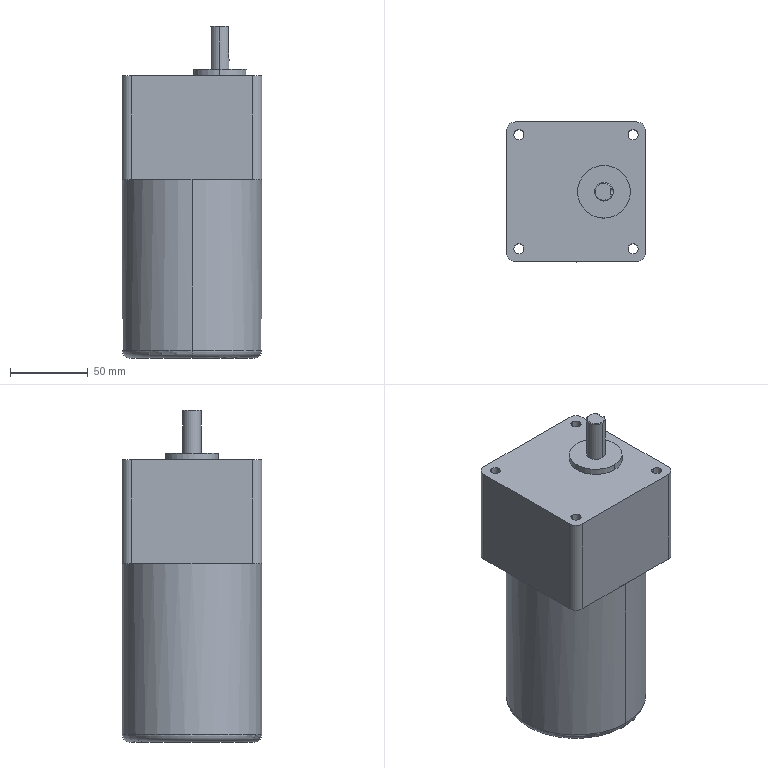Component | SolidWorks | LD101-02-5IK60Q1-C-5GN180K-1 | 1 solid | 39 faces | box 90 x 90 x 214 mm | volume 1268487 mm3 | cylinder 19 | plane 15 | cone 3 | torus 2 | commonest cylinder face diameters 6.5 x8 12 x6 34 x2 90 x2 4 x1 | material SUS304
build123d program:
from build123d import *

# Parameters (mm, degrees)
BOSS_EXTRUDE1_DEPTH        = 7
SKETCH2_R                  = 45
BOSS_EXTRUDE2_DEPTH        = 122
FILLET1_R                  = 5
BOSS_EXTRUDE3_START        = 60
BOSS_EXTRUDE3_DEPTH        = 60
SKETCH4_R                  = 17
BOSS_EXTRUDE4_DEPTH        = 4
SKETCH5_R                  = 6
BOSS_EXTRUDE5_DEPTH        = 32
CHAMFER1_SIZE              = 0.5
F_6_5_6_5_DIAMETER_HOLE1_D = 6.5
CUT_EXTRUDE2_START         = 24
CUT_EXTRUDE2_DEPTH         = 2


with BuildPart() as part:
    # Sketch1 → Boss-Extrude1 (new body)
    with BuildSketch(Plane(origin=(0, 0, 0), x_dir=(0, 0, -1), z_dir=(1, 0, 0))):
        with BuildLine():
            Line((-39, -45), (39, -45))
            ThreePointArc((39, -45), (43.243, -43.243), (45, -39))
            Line((45, -39), (45, 39))
            ThreePointArc((45, 39), (43.243, 43.243), (39, 45))
            Line((39, 45), (-39, 45))
            ThreePointArc((-39, 45), (-43.243, 43.243), (-45, 39))
            Line((-45, 39), (-45, -39))
            ThreePointArc((-45, -39), (-43.243, -43.243), (-39, -45))
        make_face()
    extrude(amount=-BOSS_EXTRUDE1_DEPTH)

    # Sketch2 → Boss-Extrude2 (add)
    with BuildSketch(Plane(origin=(0, 0, 0), x_dir=(0, 0, -1), z_dir=(1, 0, 0))):
        Circle(SKETCH2_R)
    extrude(amount=-BOSS_EXTRUDE2_DEPTH)

    # Fillet1
    fillet1_edges = [part.edges().sort_by_distance(p)[0] for p in [
        (-122, 0, 45),
    ]]
    fillet(fillet1_edges, radius=FILLET1_R)

    # Sketch3 → Boss-Extrude3 (add)
    with BuildSketch(Plane(origin=(0, 0, 0), x_dir=(0, 0, -1), z_dir=(1, 0, 0)).offset(BOSS_EXTRUDE3_START)):
        with BuildLine():
            Line((45, -39), (45, 39))
            ThreePointArc((45, 39), (43.243, 43.243), (39, 45))
            Line((39, 45), (-39, 45))
            ThreePointArc((-39, 45), (-43.243, 43.243), (-45, 39))
            Line((-45, 39), (-45, -39))
            ThreePointArc((-45, -39), (-43.243, -43.243), (-39, -45))
            Line((-39, -45), (39, -45))
            ThreePointArc((39, -45), (43.243, -43.243), (45, -39))
        make_face()
    extrude(amount=-BOSS_EXTRUDE3_DEPTH)

    # Sketch4 → Boss-Extrude4 (add)
    with BuildSketch(Plane(origin=(60, 0, 0), x_dir=(0, 0, -1), z_dir=(1, 0, 0))):
        with Locations((0, 18)):
            Circle(SKETCH4_R)
    extrude(amount=BOSS_EXTRUDE4_DEPTH)

    # Sketch5 → Boss-Extrude5 (add)
    with BuildSketch(Plane(origin=(60, 0, 0), x_dir=(0, 0, -1), z_dir=(1, 0, 0))):
        with Locations((0, 18)):
            Circle(SKETCH5_R)
    extrude(amount=BOSS_EXTRUDE5_DEPTH)

    # Chamfer1
    chamfer1_edges = [part.edges().sort_by_distance(p)[0] for p in [
        (92, 18, 6),
    ]]
    chamfer(chamfer1_edges, length=CHAMFER1_SIZE)

    # 6.5 _6.5_ Diameter Hole1 (through all)
    with Locations(Plane(origin=(60, 0, 0), x_dir=(0, 0, -1), z_dir=(1, 0, 0))):
        with Locations((36.77, 36.77), (36.77, -36.77), (-36.77, -36.77), (-36.77, 36.77)):
            Hole(F_6_5_6_5_DIAMETER_HOLE1_D / 2)

    # Sketch12 → Cut-Extrude2 (cut)
    with BuildSketch(Plane(origin=(0, 0, 0), x_dir=(1, 0, 0), z_dir=(0, 1, 0)).offset(CUT_EXTRUDE2_START)):
        with BuildLine():
            Line((92, -2), (72, -2))
            ThreePointArc((72, -2), (70, 0), (72, 2))
            Line((72, 2), (92, 2))
            ThreePointArc((92, 2), (94, 0), (92, -2))
        make_face()
    extrude(amount=-CUT_EXTRUDE2_DEPTH, mode=Mode.SUBTRACT)


solid = part.part

# Placed as in the assembly
solid = solid.moved(Location((229.211, -311.897, 223.257), (-90, 0, -90)))